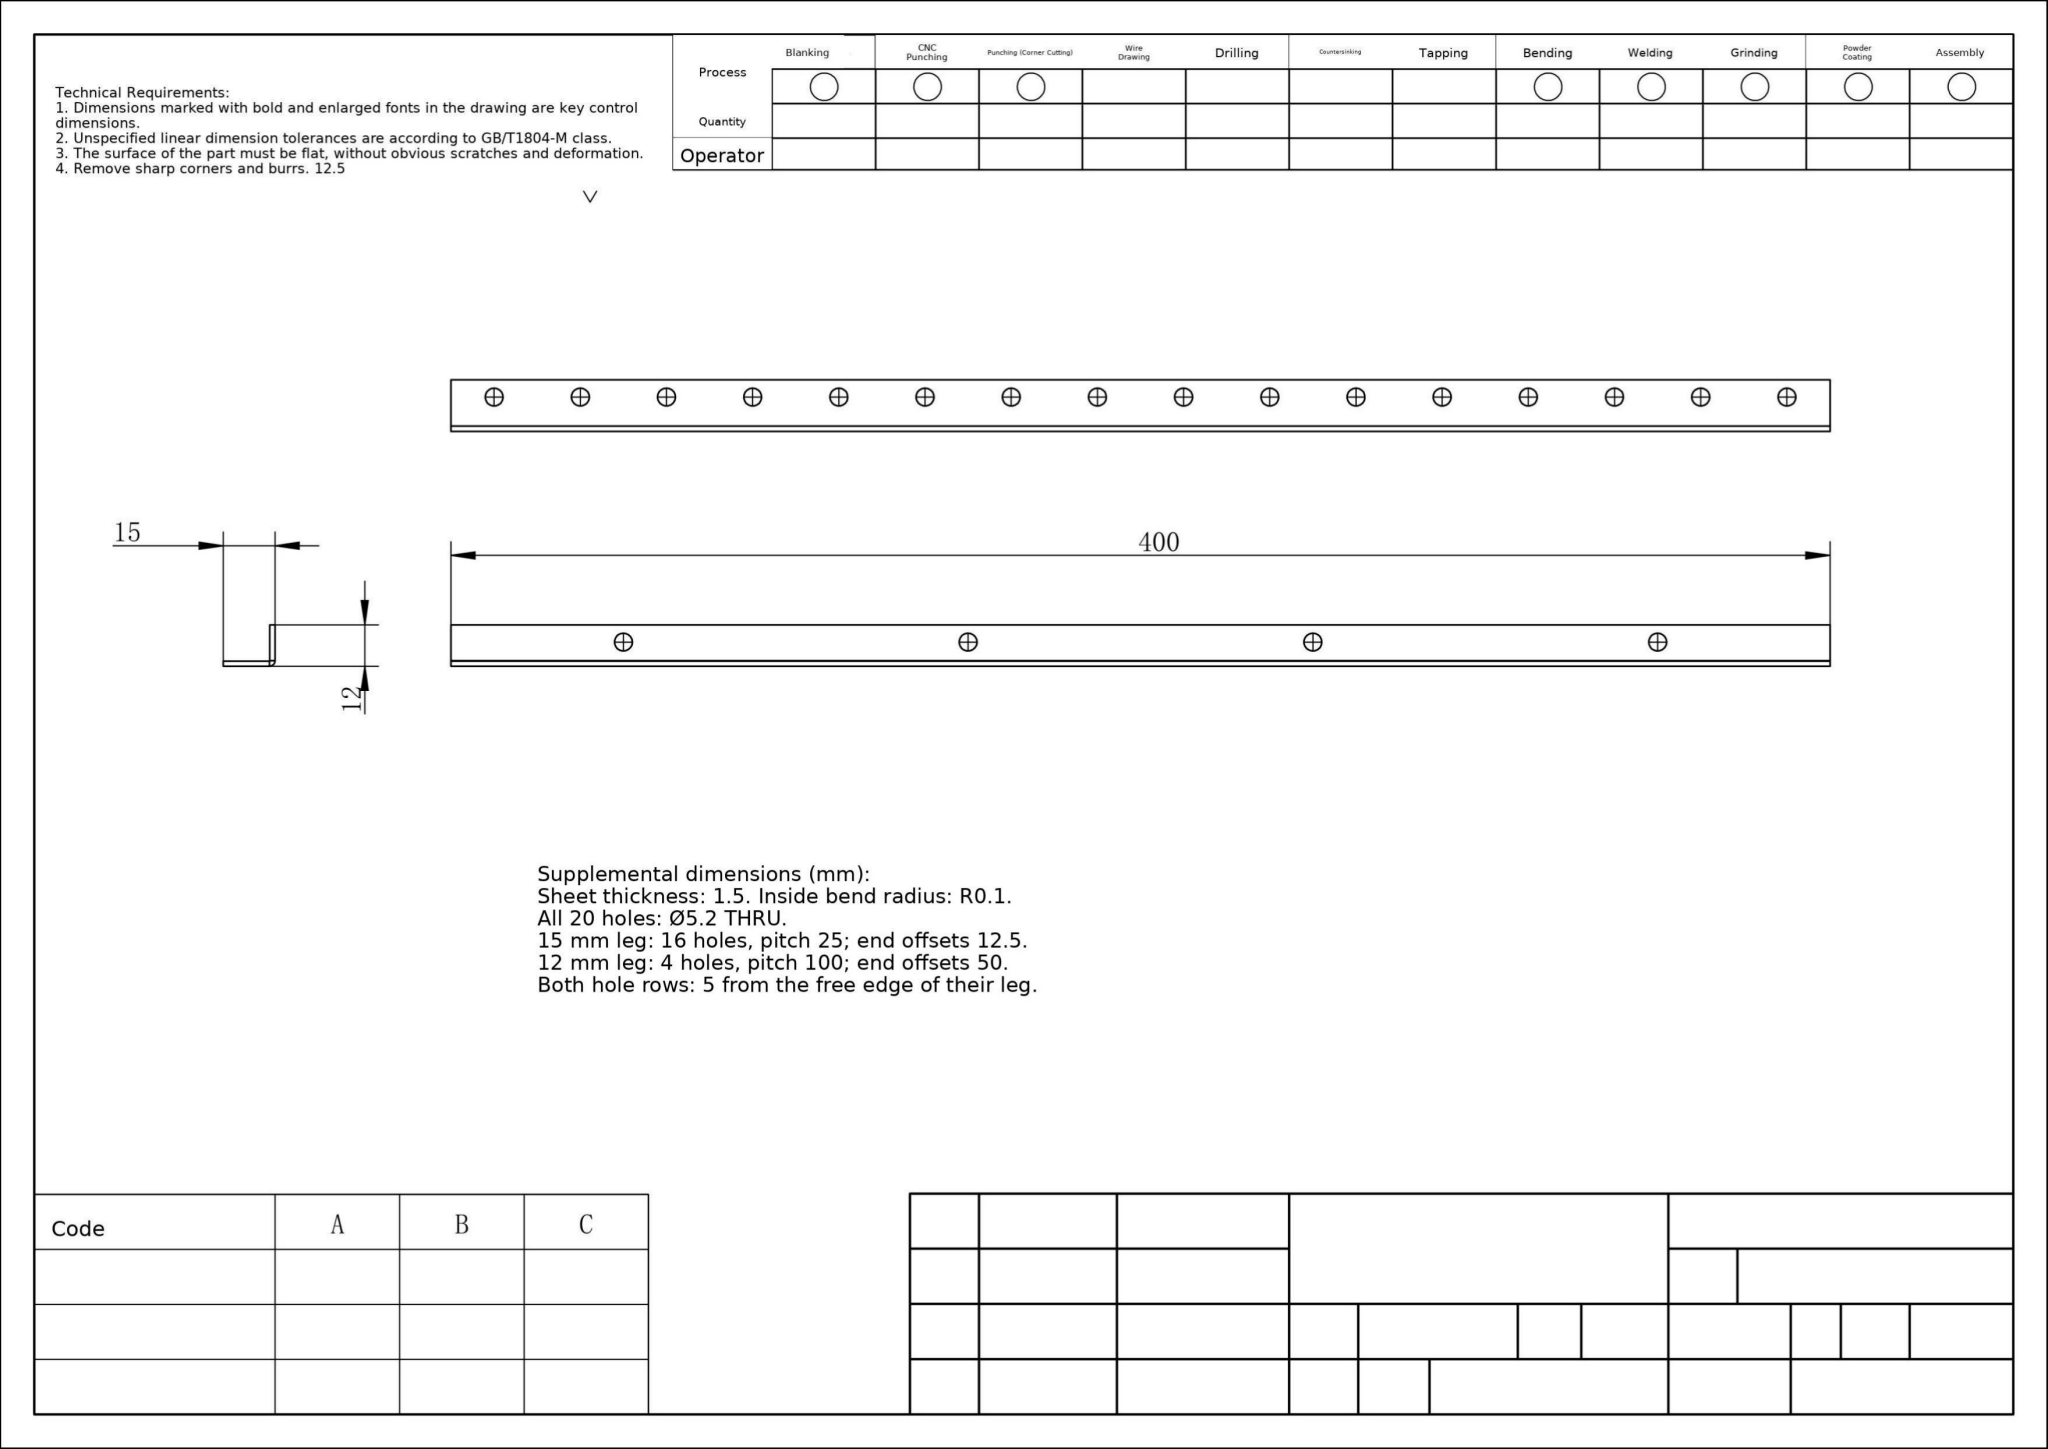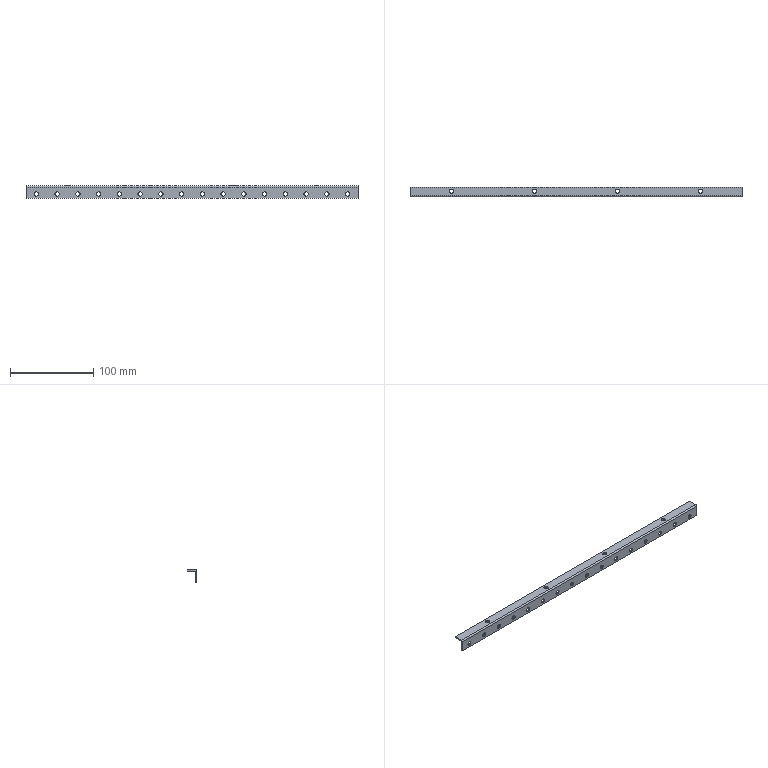Part | NX | mm | Perforated L-Shaped Mounting Rail | 1 solid | 54 faces | box 400 x 12 x 15 mm | volume 14444 mm3 | cylinder 42 | plane 12 | commonest cylinder face diameters 5.2 x40 0.2 x1 3.2 x1